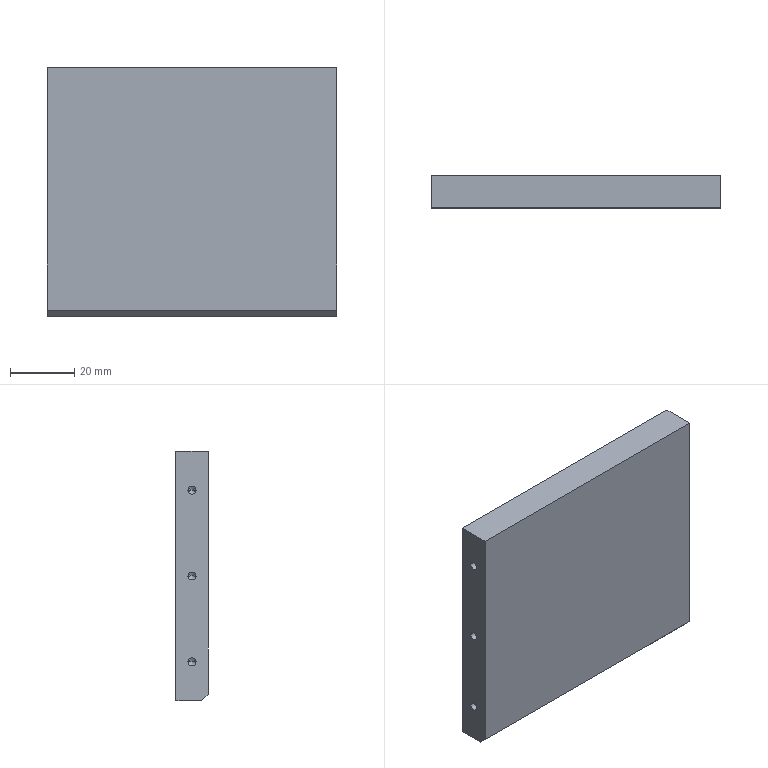Component | SolidWorks | 170423A4-SafetyPowerProbeFixingPlate4-1 | 1 solid | 31 faces | box 90 x 10 x 77.5 mm | volume 69312 mm3 | cylinder 12 | cone 12 | plane 7 | commonest cylinder face diameters 2.5 x12
build123d program:
from build123d import *

# Parameters (mm, degrees)
SKETCH1_W             = 90
SKETCH1_H             = 77.5
BOSS_EXTRUDE1_DEPTH   = 10
M3_TAPPED_HOLE1_D     = 2.5
M3_TAPPED_HOLE1_DEPTH = 8.5
M3_TAPPED_HOLE1_TIP   = 0.7511
M3_TAPPED_HOLE2_D     = 2.5
M3_TAPPED_HOLE2_DEPTH = 8.5
M3_TAPPED_HOLE2_TIP   = 0.7511
CHAMFER1_SIZE         = 2


with BuildPart() as part:
    # Sketch1 → Boss-Extrude1 (new body)
    with BuildSketch(Plane.XY):
        Rectangle(SKETCH1_W, SKETCH1_H)
    extrude(amount=BOSS_EXTRUDE1_DEPTH)

    # M3 Tapped Hole1
    with Locations(Plane(origin=(45, 0, 0), x_dir=(0, 0, -1), z_dir=(1, 0, 0))):
        with Locations((-5, 26.75), (-5, -26.75), (-5, 0)):
            Hole(M3_TAPPED_HOLE1_D / 2, depth=M3_TAPPED_HOLE1_DEPTH)
            with Locations((0, 0, -(M3_TAPPED_HOLE1_DEPTH + M3_TAPPED_HOLE1_TIP / 2))):  # 118° drill point
                Cone(0, M3_TAPPED_HOLE1_D / 2, M3_TAPPED_HOLE1_TIP, mode=Mode.SUBTRACT)

    # M3 Tapped Hole2
    with Locations(Plane.ZY.offset(45)):
        with Locations((5, 26.75), (5, 0), (5, -26.75)):
            Hole(M3_TAPPED_HOLE2_D / 2, depth=M3_TAPPED_HOLE2_DEPTH)
            with Locations((0, 0, -(M3_TAPPED_HOLE2_DEPTH + M3_TAPPED_HOLE2_TIP / 2))):  # 118° drill point
                Cone(0, M3_TAPPED_HOLE2_D / 2, M3_TAPPED_HOLE2_TIP, mode=Mode.SUBTRACT)

    # Chamfer1
    chamfer1_edges = [part.edges().sort_by_distance(p)[0] for p in [
        (0, 38.75, 10),
    ]]
    chamfer(chamfer1_edges, length=CHAMFER1_SIZE)


solid = part.part

# Placed as in the assembly
solid = solid.moved(Location((28.687, -15.611, -40.824), (90, 0, -180)))
STEP:
#1=CARTESIAN_POINT('',(2.566,-0.7622,-2.66));
#2=VERTEX_POINT('',#1);
#3=CARTESIAN_POINT('',(2.566,-0.8607,-2.66));
#4=VERTEX_POINT('',#3);
#5=CARTESIAN_POINT('',(2.566,-0.8115,-2.66));
#6=DIRECTION('',(1.,0.,0.));
#7=DIRECTION('',(0.,-1.,0.));
#8=AXIS2_PLACEMENT_3D('',#5,#6,#7);
#9=CIRCLE('',#8,0.04921);
#10=EDGE_CURVE('',#2,#4,#9,.T.);
#11=ORIENTED_EDGE('',*,*,#10,.F.);
#12=CARTESIAN_POINT('',(2.901,-0.7622,-2.66));
#13=VERTEX_POINT('',#12);
#14=CARTESIAN_POINT('',(2.901,-0.7622,-2.66));
#15=DIRECTION('',(1.,0.,0.));
#16=VECTOR('',#15,39.37);
#17=LINE('',#14,#16);
#18=EDGE_CURVE('',#2,#13,#17,.T.);
#19=ORIENTED_EDGE('',*,*,#18,.T.);
#20=CARTESIAN_POINT('',(2.901,-0.8607,-2.66));
#21=VERTEX_POINT('',#20);
#22=CARTESIAN_POINT('',(2.901,-0.8115,-2.66));
#23=DIRECTION('',(1.,0.,0.));
#24=DIRECTION('',(0.,-1.,0.));
#25=AXIS2_PLACEMENT_3D('',#22,#23,#24);
#26=CIRCLE('',#25,0.04921);
#27=EDGE_CURVE('',#13,#21,#26,.T.);
#28=ORIENTED_EDGE('',*,*,#27,.T.);
#29=CARTESIAN_POINT('',(2.901,-0.8607,-2.66));
#30=DIRECTION('',(1.,0.,0.));
#31=VECTOR('',#30,39.37);
#32=LINE('',#29,#31);
#33=EDGE_CURVE('',#4,#21,#32,.T.);
#34=ORIENTED_EDGE('',*,*,#33,.F.);
#35=EDGE_LOOP('',(#11,#19,#28,#34));
#36=FACE_OUTER_BOUND('',#35,.T.);
#37=CARTESIAN_POINT('',(2.901,-0.8115,-2.66));
#38=DIRECTION('',(1.,0.,0.));
#39=DIRECTION('',(0.,-1.,0.));
#40=AXIS2_PLACEMENT_3D('',#37,#38,#39);
#41=CYLINDRICAL_SURFACE('',#40,0.04921);
#42=ADVANCED_FACE('',(#36),#41,.F.);
#43=CARTESIAN_POINT('',(2.537,-0.8115,-2.66));
#44=VERTEX_POINT('',#43);
#45=CARTESIAN_POINT('',(2.566,-0.8607,-2.66));
#46=DIRECTION('',(0.515,-0.8572,0.));
#47=VECTOR('',#46,39.37);
#48=LINE('',#45,#47);
#49=EDGE_CURVE('',#44,#4,#48,.T.);
#50=ORIENTED_EDGE('',*,*,#49,.F.);
#51=CARTESIAN_POINT('',(2.566,-0.7622,-2.66));
#52=DIRECTION('',(0.515,0.8572,-0.));
#53=VECTOR('',#52,39.37);
#54=LINE('',#51,#53);
#55=EDGE_CURVE('',#44,#2,#54,.T.);
#56=ORIENTED_EDGE('',*,*,#55,.T.);
#57=ORIENTED_EDGE('',*,*,#10,.T.);
#58=EDGE_LOOP('',(#50,#56,#57));
#59=FACE_OUTER_BOUND('',#58,.T.);
#60=CARTESIAN_POINT('',(2.566,-0.8115,-2.66));
#61=DIRECTION('',(1.,0.,0.));
#62=DIRECTION('',(0.,-1.,0.));
#63=AXIS2_PLACEMENT_3D('',#60,#61,#62);
#64=CONICAL_SURFACE('',#63,0.04921,1.03);
#65=ADVANCED_FACE('',(#59),#64,.F.);
#66=CARTESIAN_POINT('',(2.566,-0.7622,-1.607));
#67=VERTEX_POINT('',#66);
#68=CARTESIAN_POINT('',(2.566,-0.8607,-1.607));
#69=VERTEX_POINT('',#68);
#70=CARTESIAN_POINT('',(2.566,-0.8115,-1.607));
#71=DIRECTION('',(1.,0.,0.));
#72=DIRECTION('',(0.,-1.,0.));
#73=AXIS2_PLACEMENT_3D('',#70,#71,#72);
#74=CIRCLE('',#73,0.04921);
#75=EDGE_CURVE('',#67,#69,#74,.T.);
#76=ORIENTED_EDGE('',*,*,#75,.F.);
#77=CARTESIAN_POINT('',(2.901,-0.7622,-1.607));
#78=VERTEX_POINT('',#77);
#79=CARTESIAN_POINT('',(2.901,-0.7622,-1.607));
#80=DIRECTION('',(1.,0.,0.));
#81=VECTOR('',#80,39.37);
#82=LINE('',#79,#81);
#83=EDGE_CURVE('',#67,#78,#82,.T.);
#84=ORIENTED_EDGE('',*,*,#83,.T.);
#85=CARTESIAN_POINT('',(2.901,-0.8607,-1.607));
#86=VERTEX_POINT('',#85);
#87=CARTESIAN_POINT('',(2.901,-0.8115,-1.607));
#88=DIRECTION('',(1.,0.,0.));
#89=DIRECTION('',(0.,-1.,0.));
#90=AXIS2_PLACEMENT_3D('',#87,#88,#89);
#91=CIRCLE('',#90,0.04921);
#92=EDGE_CURVE('',#78,#86,#91,.T.);
#93=ORIENTED_EDGE('',*,*,#92,.T.);
#94=CARTESIAN_POINT('',(2.901,-0.8607,-1.607));
#95=DIRECTION('',(1.,0.,0.));
#96=VECTOR('',#95,39.37);
#97=LINE('',#94,#96);
#98=EDGE_CURVE('',#69,#86,#97,.T.);
#99=ORIENTED_EDGE('',*,*,#98,.F.);
#100=EDGE_LOOP('',(#76,#84,#93,#99));
#101=FACE_OUTER_BOUND('',#100,.T.);
#102=CARTESIAN_POINT('',(2.901,-0.8115,-1.607));
#103=DIRECTION('',(1.,0.,0.));
#104=DIRECTION('',(0.,-1.,0.));
#105=AXIS2_PLACEMENT_3D('',#102,#103,#104);
#106=CYLINDRICAL_SURFACE('',#105,0.04921);
#107=ADVANCED_FACE('',(#101),#106,.F.);
#108=CARTESIAN_POINT('',(2.537,-0.8115,-1.607));
#109=VERTEX_POINT('',#108);
#110=CARTESIAN_POINT('',(2.566,-0.8607,-1.607));
#111=DIRECTION('',(0.515,-0.8572,0.));
#112=VECTOR('',#111,39.37);
#113=LINE('',#110,#112);
#114=EDGE_CURVE('',#109,#69,#113,.T.);
#115=ORIENTED_EDGE('',*,*,#114,.F.);
#116=CARTESIAN_POINT('',(2.566,-0.7622,-1.607));
#117=DIRECTION('',(0.515,0.8572,-0.));
#118=VECTOR('',#117,39.37);
#119=LINE('',#116,#118);
#120=EDGE_CURVE('',#109,#67,#119,.T.);
#121=ORIENTED_EDGE('',*,*,#120,.T.);
#122=ORIENTED_EDGE('',*,*,#75,.T.);
#123=EDGE_LOOP('',(#115,#121,#122));
#124=FACE_OUTER_BOUND('',#123,.T.);
#125=CARTESIAN_POINT('',(2.566,-0.8115,-1.607));
#126=DIRECTION('',(1.,0.,0.));
#127=DIRECTION('',(0.,-1.,0.));
#128=AXIS2_PLACEMENT_3D('',#125,#126,#127);
#129=CONICAL_SURFACE('',#128,0.04921,1.03);
#130=ADVANCED_FACE('',(#124),#129,.F.);
#131=CARTESIAN_POINT('',(2.566,-0.7622,-0.5541));
#132=VERTEX_POINT('',#131);
#133=CARTESIAN_POINT('',(2.566,-0.8607,-0.5541));
#134=VERTEX_POINT('',#133);
#135=CARTESIAN_POINT('',(2.566,-0.8115,-0.5541));
#136=DIRECTION('',(1.,0.,0.));
#137=DIRECTION('',(0.,-1.,0.));
#138=AXIS2_PLACEMENT_3D('',#135,#136,#137);
#139=CIRCLE('',#138,0.04921);
#140=EDGE_CURVE('',#132,#134,#139,.T.);
#141=ORIENTED_EDGE('',*,*,#140,.F.);
#142=CARTESIAN_POINT('',(2.901,-0.7622,-0.5541));
#143=VERTEX_POINT('',#142);
#144=CARTESIAN_POINT('',(2.901,-0.7622,-0.5541));
#145=DIRECTION('',(1.,0.,0.));
#146=VECTOR('',#145,39.37);
#147=LINE('',#144,#146);
#148=EDGE_CURVE('',#132,#143,#147,.T.);
#149=ORIENTED_EDGE('',*,*,#148,.T.);
#150=CARTESIAN_POINT('',(2.901,-0.8607,-0.5541));
#151=VERTEX_POINT('',#150);
#152=CARTESIAN_POINT('',(2.901,-0.8115,-0.5541));
#153=DIRECTION('',(1.,0.,0.));
#154=DIRECTION('',(0.,-1.,0.));
#155=AXIS2_PLACEMENT_3D('',#152,#153,#154);
#156=CIRCLE('',#155,0.04921);
#157=EDGE_CURVE('',#143,#151,#156,.T.);
#158=ORIENTED_EDGE('',*,*,#157,.T.);
#159=CARTESIAN_POINT('',(2.901,-0.8607,-0.5541));
#160=DIRECTION('',(1.,0.,0.));
#161=VECTOR('',#160,39.37);
#162=LINE('',#159,#161);
#163=EDGE_CURVE('',#134,#151,#162,.T.);
#164=ORIENTED_EDGE('',*,*,#163,.F.);
#165=EDGE_LOOP('',(#141,#149,#158,#164));
#166=FACE_OUTER_BOUND('',#165,.T.);
#167=CARTESIAN_POINT('',(2.901,-0.8115,-0.5541));
#168=DIRECTION('',(1.,0.,0.));
#169=DIRECTION('',(0.,-1.,0.));
#170=AXIS2_PLACEMENT_3D('',#167,#168,#169);
#171=CYLINDRICAL_SURFACE('',#170,0.04921);
#172=ADVANCED_FACE('',(#166),#171,.F.);
#173=CARTESIAN_POINT('',(2.537,-0.8115,-0.5541));
#174=VERTEX_POINT('',#173);
#175=CARTESIAN_POINT('',(2.566,-0.8607,-0.5541));
#176=DIRECTION('',(0.515,-0.8572,0.));
#177=VECTOR('',#176,39.37);
#178=LINE('',#175,#177);
#179=EDGE_CURVE('',#174,#134,#178,.T.);
#180=ORIENTED_EDGE('',*,*,#179,.F.);
#181=CARTESIAN_POINT('',(2.566,-0.7622,-0.5541));
#182=DIRECTION('',(0.515,0.8572,-0.));
#183=VECTOR('',#182,39.37);
#184=LINE('',#181,#183);
#185=EDGE_CURVE('',#174,#132,#184,.T.);
#186=ORIENTED_EDGE('',*,*,#185,.T.);
#187=ORIENTED_EDGE('',*,*,#140,.T.);
#188=EDGE_LOOP('',(#180,#186,#187));
#189=FACE_OUTER_BOUND('',#188,.T.);
#190=CARTESIAN_POINT('',(2.566,-0.8115,-0.5541));
#191=DIRECTION('',(1.,0.,0.));
#192=DIRECTION('',(0.,-1.,0.));
#193=AXIS2_PLACEMENT_3D('',#190,#191,#192);
#194=CONICAL_SURFACE('',#193,0.04921,1.03);
#195=ADVANCED_FACE('',(#189),#194,.F.);
#196=CARTESIAN_POINT('',(-0.3076,-0.8607,-0.5541));
#197=VERTEX_POINT('',#196);
#198=CARTESIAN_POINT('',(-0.3076,-0.7622,-0.5541));
#199=VERTEX_POINT('',#198);
#200=CARTESIAN_POINT('',(-0.3076,-0.8115,-0.5541));
#201=DIRECTION('',(-1.,-0.,-0.));
#202=DIRECTION('',(0.,1.,0.));
#203=AXIS2_PLACEMENT_3D('',#200,#201,#202);
#204=CIRCLE('',#203,0.04921);
#205=EDGE_CURVE('',#197,#199,#204,.T.);
#206=ORIENTED_EDGE('',*,*,#205,.F.);
#207=CARTESIAN_POINT('',(-0.6423,-0.8607,-0.5541));
#208=VERTEX_POINT('',#207);
#209=CARTESIAN_POINT('',(-0.6423,-0.8607,-0.5541));
#210=DIRECTION('',(-1.,-0.,-0.));
#211=VECTOR('',#210,39.37);
#212=LINE('',#209,#211);
#213=EDGE_CURVE('',#197,#208,#212,.T.);
#214=ORIENTED_EDGE('',*,*,#213,.T.);
#215=CARTESIAN_POINT('',(-0.6423,-0.7622,-0.5541));
#216=VERTEX_POINT('',#215);
#217=CARTESIAN_POINT('',(-0.6423,-0.8115,-0.5541));
#218=DIRECTION('',(-1.,-0.,-0.));
#219=DIRECTION('',(0.,1.,0.));
#220=AXIS2_PLACEMENT_3D('',#217,#218,#219);
#221=CIRCLE('',#220,0.04921);
#222=EDGE_CURVE('',#208,#216,#221,.T.);
#223=ORIENTED_EDGE('',*,*,#222,.T.);
#224=CARTESIAN_POINT('',(-0.6423,-0.7622,-0.5541));
#225=DIRECTION('',(-1.,-0.,-0.));
#226=VECTOR('',#225,39.37);
#227=LINE('',#224,#226);
#228=EDGE_CURVE('',#199,#216,#227,.T.);
#229=ORIENTED_EDGE('',*,*,#228,.F.);
#230=EDGE_LOOP('',(#206,#214,#223,#229));
#231=FACE_OUTER_BOUND('',#230,.T.);
#232=CARTESIAN_POINT('',(-0.6423,-0.8115,-0.5541));
#233=DIRECTION('',(-1.,-0.,-0.));
#234=DIRECTION('',(0.,1.,0.));
#235=AXIS2_PLACEMENT_3D('',#232,#233,#234);
#236=CYLINDRICAL_SURFACE('',#235,0.04921);
#237=ADVANCED_FACE('',(#231),#236,.F.);
#238=CARTESIAN_POINT('',(-0.278,-0.8115,-0.5541));
#239=VERTEX_POINT('',#238);
#240=CARTESIAN_POINT('',(-0.3076,-0.7622,-0.5541));
#241=DIRECTION('',(-0.515,0.8572,-0.));
#242=VECTOR('',#241,39.37);
#243=LINE('',#240,#242);
#244=EDGE_CURVE('',#239,#199,#243,.T.);
#245=ORIENTED_EDGE('',*,*,#244,.F.);
#246=CARTESIAN_POINT('',(-0.3076,-0.8607,-0.5541));
#247=DIRECTION('',(-0.515,-0.8572,-0.));
#248=VECTOR('',#247,39.37);
#249=LINE('',#246,#248);
#250=EDGE_CURVE('',#239,#197,#249,.T.);
#251=ORIENTED_EDGE('',*,*,#250,.T.);
#252=ORIENTED_EDGE('',*,*,#205,.T.);
#253=EDGE_LOOP('',(#245,#251,#252));
#254=FACE_OUTER_BOUND('',#253,.T.);
#255=CARTESIAN_POINT('',(-0.3076,-0.8115,-0.5541));
#256=DIRECTION('',(-1.,-0.,-0.));
#257=DIRECTION('',(0.,1.,0.));
#258=AXIS2_PLACEMENT_3D('',#255,#256,#257);
#259=CONICAL_SURFACE('',#258,0.04921,1.03);
#260=ADVANCED_FACE('',(#254),#259,.F.);
#261=CARTESIAN_POINT('',(-0.3076,-0.8607,-1.607));
#262=VERTEX_POINT('',#261);
#263=CARTESIAN_POINT('',(-0.3076,-0.7622,-1.607));
#264=VERTEX_POINT('',#263);
#265=CARTESIAN_POINT('',(-0.3076,-0.8115,-1.607));
#266=DIRECTION('',(-1.,-0.,-0.));
#267=DIRECTION('',(0.,1.,0.));
#268=AXIS2_PLACEMENT_3D('',#265,#266,#267);
#269=CIRCLE('',#268,0.04921);
#270=EDGE_CURVE('',#262,#264,#269,.T.);
#271=ORIENTED_EDGE('',*,*,#270,.F.);
#272=CARTESIAN_POINT('',(-0.6423,-0.8607,-1.607));
#273=VERTEX_POINT('',#272);
#274=CARTESIAN_POINT('',(-0.6423,-0.8607,-1.607));
#275=DIRECTION('',(-1.,-0.,-0.));
#276=VECTOR('',#275,39.37);
#277=LINE('',#274,#276);
#278=EDGE_CURVE('',#262,#273,#277,.T.);
#279=ORIENTED_EDGE('',*,*,#278,.T.);
#280=CARTESIAN_POINT('',(-0.6423,-0.7622,-1.607));
#281=VERTEX_POINT('',#280);
#282=CARTESIAN_POINT('',(-0.6423,-0.8115,-1.607));
#283=DIRECTION('',(-1.,-0.,-0.));
#284=DIRECTION('',(0.,1.,0.));
#285=AXIS2_PLACEMENT_3D('',#282,#283,#284);
#286=CIRCLE('',#285,0.04921);
#287=EDGE_CURVE('',#273,#281,#286,.T.);
#288=ORIENTED_EDGE('',*,*,#287,.T.);
#289=CARTESIAN_POINT('',(-0.6423,-0.7622,-1.607));
#290=DIRECTION('',(-1.,-0.,-0.));
#291=VECTOR('',#290,39.37);
#292=LINE('',#289,#291);
#293=EDGE_CURVE('',#264,#281,#292,.T.);
#294=ORIENTED_EDGE('',*,*,#293,.F.);
#295=EDGE_LOOP('',(#271,#279,#288,#294));
#296=FACE_OUTER_BOUND('',#295,.T.);
#297=CARTESIAN_POINT('',(-0.6423,-0.8115,-1.607));
#298=DIRECTION('',(-1.,-0.,-0.));
#299=DIRECTION('',(0.,1.,0.));
#300=AXIS2_PLACEMENT_3D('',#297,#298,#299);
#301=CYLINDRICAL_SURFACE('',#300,0.04921);
#302=ADVANCED_FACE('',(#296),#301,.F.);
#303=CARTESIAN_POINT('',(-0.278,-0.8115,-1.607));
#304=VERTEX_POINT('',#303);
#305=CARTESIAN_POINT('',(-0.3076,-0.7622,-1.607));
#306=DIRECTION('',(-0.515,0.8572,-0.));
#307=VECTOR('',#306,39.37);
#308=LINE('',#305,#307);
#309=EDGE_CURVE('',#304,#264,#308,.T.);
#310=ORIENTED_EDGE('',*,*,#309,.F.);
#311=CARTESIAN_POINT('',(-0.3076,-0.8607,-1.607));
#312=DIRECTION('',(-0.515,-0.8572,-0.));
#313=VECTOR('',#312,39.37);
#314=LINE('',#311,#313);
#315=EDGE_CURVE('',#304,#262,#314,.T.);
#316=ORIENTED_EDGE('',*,*,#315,.T.);
#317=ORIENTED_EDGE('',*,*,#270,.T.);
#318=EDGE_LOOP('',(#310,#316,#317));
#319=FACE_OUTER_BOUND('',#318,.T.);
#320=CARTESIAN_POINT('',(-0.3076,-0.8115,-1.607));
#321=DIRECTION('',(-1.,-0.,-0.));
#322=DIRECTION('',(0.,1.,0.));
#323=AXIS2_PLACEMENT_3D('',#320,#321,#322);
#324=CONICAL_SURFACE('',#323,0.04921,1.03);
#325=ADVANCED_FACE('',(#319),#324,.F.);
#326=CARTESIAN_POINT('',(-0.3076,-0.8607,-2.66));
#327=VERTEX_POINT('',#326);
#328=CARTESIAN_POINT('',(-0.3076,-0.7622,-2.66));
#329=VERTEX_POINT('',#328);
#330=CARTESIAN_POINT('',(-0.3076,-0.8115,-2.66));
#331=DIRECTION('',(-1.,-0.,-0.));
#332=DIRECTION('',(0.,1.,0.));
#333=AXIS2_PLACEMENT_3D('',#330,#331,#332);
#334=CIRCLE('',#333,0.04921);
#335=EDGE_CURVE('',#327,#329,#334,.T.);
#336=ORIENTED_EDGE('',*,*,#335,.F.);
#337=CARTESIAN_POINT('',(-0.6423,-0.8607,-2.66));
#338=VERTEX_POINT('',#337);
#339=CARTESIAN_POINT('',(-0.6423,-0.8607,-2.66));
#340=DIRECTION('',(-1.,-0.,-0.));
#341=VECTOR('',#340,39.37);
#342=LINE('',#339,#341);
#343=EDGE_CURVE('',#327,#338,#342,.T.);
#344=ORIENTED_EDGE('',*,*,#343,.T.);
#345=CARTESIAN_POINT('',(-0.6423,-0.7622,-2.66));
#346=VERTEX_POINT('',#345);
#347=CARTESIAN_POINT('',(-0.6423,-0.8115,-2.66));
#348=DIRECTION('',(-1.,-0.,-0.));
#349=DIRECTION('',(0.,1.,0.));
#350=AXIS2_PLACEMENT_3D('',#347,#348,#349);
#351=CIRCLE('',#350,0.04921);
#352=EDGE_CURVE('',#338,#346,#351,.T.);
#353=ORIENTED_EDGE('',*,*,#352,.T.);
#354=CARTESIAN_POINT('',(-0.6423,-0.7622,-2.66));
#355=DIRECTION('',(-1.,-0.,-0.));
#356=VECTOR('',#355,39.37);
#357=LINE('',#354,#356);
#358=EDGE_CURVE('',#329,#346,#357,.T.);
#359=ORIENTED_EDGE('',*,*,#358,.F.);
#360=EDGE_LOOP('',(#336,#344,#353,#359));
#361=FACE_OUTER_BOUND('',#360,.T.);
#362=CARTESIAN_POINT('',(-0.6423,-0.8115,-2.66));
#363=DIRECTION('',(-1.,-0.,-0.));
#364=DIRECTION('',(0.,1.,0.));
#365=AXIS2_PLACEMENT_3D('',#362,#363,#364);
#366=CYLINDRICAL_SURFACE('',#365,0.04921);
#367=ADVANCED_FACE('',(#361),#366,.F.);
#368=CARTESIAN_POINT('',(-0.278,-0.8115,-2.66));
#369=VERTEX_POINT('',#368);
#370=CARTESIAN_POINT('',(-0.3076,-0.7622,-2.66));
#371=DIRECTION('',(-0.515,0.8572,-0.));
#372=VECTOR('',#371,39.37);
#373=LINE('',#370,#372);
#374=EDGE_CURVE('',#369,#329,#373,.T.);
#375=ORIENTED_EDGE('',*,*,#374,.F.);
#376=CARTESIAN_POINT('',(-0.3076,-0.8607,-2.66));
#377=DIRECTION('',(-0.515,-0.8572,-0.));
#378=VECTOR('',#377,39.37);
#379=LINE('',#376,#378);
#380=EDGE_CURVE('',#369,#327,#379,.T.);
#381=ORIENTED_EDGE('',*,*,#380,.T.);
#382=ORIENTED_EDGE('',*,*,#335,.T.);
#383=EDGE_LOOP('',(#375,#381,#382));
#384=FACE_OUTER_BOUND('',#383,.T.);
#385=CARTESIAN_POINT('',(-0.3076,-0.8115,-2.66));
#386=DIRECTION('',(-1.,-0.,-0.));
#387=DIRECTION('',(0.,1.,0.));
#388=AXIS2_PLACEMENT_3D('',#385,#386,#387);
#389=CONICAL_SURFACE('',#388,0.04921,1.03);
#390=ADVANCED_FACE('',(#384),#389,.F.);
#391=CARTESIAN_POINT('',(-0.6423,-0.8115,-0.5541));
#392=DIRECTION('',(-1.,-0.,-0.));
#393=DIRECTION('',(0.,1.,0.));
#394=AXIS2_PLACEMENT_3D('',#391,#392,#393);
#395=CIRCLE('',#394,0.04921);
#396=EDGE_CURVE('',#216,#208,#395,.T.);
#397=ORIENTED_EDGE('',*,*,#396,.F.);
#398=ORIENTED_EDGE('',*,*,#222,.F.);
#399=EDGE_LOOP('',(#397,#398));
#400=FACE_BOUND('',#399,.T.);
#401=CARTESIAN_POINT('',(-0.6423,-0.8115,-1.607));
#402=DIRECTION('',(-1.,-0.,-0.));
#403=DIRECTION('',(0.,1.,0.));
#404=AXIS2_PLACEMENT_3D('',#401,#402,#403);
#405=CIRCLE('',#404,0.04921);
#406=EDGE_CURVE('',#281,#273,#405,.T.);
#407=ORIENTED_EDGE('',*,*,#406,.F.);
#408=ORIENTED_EDGE('',*,*,#287,.F.);
#409=EDGE_LOOP('',(#407,#408));
#410=FACE_BOUND('',#409,.T.);
#411=CARTESIAN_POINT('',(-0.6423,-0.8115,-2.66));
#412=DIRECTION('',(-1.,-0.,-0.));
#413=DIRECTION('',(0.,1.,0.));
#414=AXIS2_PLACEMENT_3D('',#411,#412,#413);
#415=CIRCLE('',#414,0.04921);
#416=EDGE_CURVE('',#346,#338,#415,.T.);
#417=ORIENTED_EDGE('',*,*,#416,.F.);
#418=ORIENTED_EDGE('',*,*,#352,.F.);
#419=EDGE_LOOP('',(#417,#418));
#420=FACE_BOUND('',#419,.T.);
#421=CARTESIAN_POINT('',(-0.6423,-0.9296,-3.133));
#422=VERTEX_POINT('',#421);
#423=CARTESIAN_POINT('',(-0.6423,-0.6146,-3.133));
#424=VERTEX_POINT('',#423);
#425=CARTESIAN_POINT('',(-0.6423,-1.008,-3.133));
#426=DIRECTION('',(-0.,1.,0.));
#427=VECTOR('',#426,39.37);
#428=LINE('',#425,#427);
#429=EDGE_CURVE('',#422,#424,#428,.T.);
#430=ORIENTED_EDGE('',*,*,#429,.F.);
#431=CARTESIAN_POINT('',(-0.6423,-1.008,-3.054));
#432=VERTEX_POINT('',#431);
#433=CARTESIAN_POINT('',(-0.6423,-1.008,-3.054));
#434=DIRECTION('',(-0.,-0.7071,0.7071));
#435=VECTOR('',#434,39.37);
#436=LINE('',#433,#435);
#437=EDGE_CURVE('',#422,#432,#436,.T.);
#438=ORIENTED_EDGE('',*,*,#437,.T.);
#439=CARTESIAN_POINT('',(-0.6423,-1.008,-0.08165));
#440=VERTEX_POINT('',#439);
#441=CARTESIAN_POINT('',(-0.6423,-1.008,-3.133));
#442=DIRECTION('',(0.,-0.,-1.));
#443=VECTOR('',#442,39.37);
#444=LINE('',#441,#443);
#445=EDGE_CURVE('',#440,#432,#444,.T.);
#446=ORIENTED_EDGE('',*,*,#445,.F.);
#447=CARTESIAN_POINT('',(-0.6423,-0.6146,-0.08165));
#448=VERTEX_POINT('',#447);
#449=CARTESIAN_POINT('',(-0.6423,-1.008,-0.08165));
#450=DIRECTION('',(-0.,1.,0.));
#451=VECTOR('',#450,39.37);
#452=LINE('',#449,#451);
#453=EDGE_CURVE('',#440,#448,#452,.T.);
#454=ORIENTED_EDGE('',*,*,#453,.T.);
#455=CARTESIAN_POINT('',(-0.6423,-0.6146,-3.133));
#456=DIRECTION('',(0.,-0.,-1.));
#457=VECTOR('',#456,39.37);
#458=LINE('',#455,#457);
#459=EDGE_CURVE('',#448,#424,#458,.T.);
#460=ORIENTED_EDGE('',*,*,#459,.T.);
#461=EDGE_LOOP('',(#430,#438,#446,#454,#460));
#462=FACE_OUTER_BOUND('',#461,.T.);
#463=CARTESIAN_POINT('',(-0.6423,-1.008,-3.133));
#464=DIRECTION('',(1.,0.,0.));
#465=DIRECTION('',(-0.,0.,1.));
#466=AXIS2_PLACEMENT_3D('',#463,#464,#465);
#467=PLANE('',#466);
#468=ADVANCED_FACE('',(#400,#410,#420,#462),#467,.F.);
#469=CARTESIAN_POINT('',(2.901,-0.9296,-3.133));
#470=VERTEX_POINT('',#469);
#471=CARTESIAN_POINT('',(2.901,-0.6146,-3.133));
#472=VERTEX_POINT('',#471);
#473=CARTESIAN_POINT('',(2.901,-1.008,-3.133));
#474=DIRECTION('',(-0.,1.,0.));
#475=VECTOR('',#474,39.37);
#476=LINE('',#473,#475);
#477=EDGE_CURVE('',#470,#472,#476,.T.);
#478=ORIENTED_EDGE('',*,*,#477,.F.);
#479=CARTESIAN_POINT('',(-0.6423,-0.9296,-3.133));
#480=DIRECTION('',(-1.,-0.,-0.));
#481=VECTOR('',#480,39.37);
#482=LINE('',#479,#481);
#483=EDGE_CURVE('',#470,#422,#482,.T.);
#484=ORIENTED_EDGE('',*,*,#483,.T.);
#485=ORIENTED_EDGE('',*,*,#429,.T.);
#486=CARTESIAN_POINT('',(2.901,-0.6146,-3.133));
#487=DIRECTION('',(1.,0.,0.));
#488=VECTOR('',#487,39.37);
#489=LINE('',#486,#488);
#490=EDGE_CURVE('',#424,#472,#489,.T.);
#491=ORIENTED_EDGE('',*,*,#490,.T.);
#492=EDGE_LOOP('',(#478,#484,#485,#491));
#493=FACE_OUTER_BOUND('',#492,.T.);
#494=CARTESIAN_POINT('',(2.901,-1.008,-3.133));
#495=DIRECTION('',(0.,-0.,1.));
#496=DIRECTION('',(-0.,1.,0.));
#497=AXIS2_PLACEMENT_3D('',#494,#495,#496);
#498=PLANE('',#497);
#499=ADVANCED_FACE('',(#493),#498,.F.);
#500=CARTESIAN_POINT('',(2.901,-0.8115,-2.66));
#501=DIRECTION('',(1.,0.,0.));
#502=DIRECTION('',(0.,-1.,0.));
#503=AXIS2_PLACEMENT_3D('',#500,#501,#502);
#504=CIRCLE('',#503,0.04921);
#505=EDGE_CURVE('',#21,#13,#504,.T.);
#506=ORIENTED_EDGE('',*,*,#505,.F.);
#507=ORIENTED_EDGE('',*,*,#27,.F.);
#508=EDGE_LOOP('',(#506,#507));
#509=FACE_BOUND('',#508,.T.);
#510=CARTESIAN_POINT('',(2.901,-0.8115,-1.607));
#511=DIRECTION('',(1.,0.,0.));
#512=DIRECTION('',(0.,-1.,0.));
#513=AXIS2_PLACEMENT_3D('',#510,#511,#512);
#514=CIRCLE('',#513,0.04921);
#515=EDGE_CURVE('',#86,#78,#514,.T.);
#516=ORIENTED_EDGE('',*,*,#515,.F.);
#517=ORIENTED_EDGE('',*,*,#92,.F.);
#518=EDGE_LOOP('',(#516,#517));
#519=FACE_BOUND('',#518,.T.);
#520=CARTESIAN_POINT('',(2.901,-0.8115,-0.5541));
#521=DIRECTION('',(1.,0.,0.));
#522=DIRECTION('',(0.,-1.,0.));
#523=AXIS2_PLACEMENT_3D('',#520,#521,#522);
#524=CIRCLE('',#523,0.04921);
#525=EDGE_CURVE('',#151,#143,#524,.T.);
#526=ORIENTED_EDGE('',*,*,#525,.F.);
#527=ORIENTED_EDGE('',*,*,#157,.F.);
#528=EDGE_LOOP('',(#526,#527));
#529=FACE_BOUND('',#528,.T.);
#530=CARTESIAN_POINT('',(2.901,-1.008,-3.054));
#531=VERTEX_POINT('',#530);
#532=CARTESIAN_POINT('',(2.901,-1.008,-0.08165));
#533=VERTEX_POINT('',#532);
#534=CARTESIAN_POINT('',(2.901,-1.008,-3.133));
#535=DIRECTION('',(-0.,0.,1.));
#536=VECTOR('',#535,39.37);
#537=LINE('',#534,#536);
#538=EDGE_CURVE('',#531,#533,#537,.T.);
#539=ORIENTED_EDGE('',*,*,#538,.F.);
#540=CARTESIAN_POINT('',(2.901,-1.008,-3.054));
#541=DIRECTION('',(-0.,0.7071,-0.7071));
#542=VECTOR('',#541,39.37);
#543=LINE('',#540,#542);
#544=EDGE_CURVE('',#531,#470,#543,.T.);
#545=ORIENTED_EDGE('',*,*,#544,.T.);
#546=ORIENTED_EDGE('',*,*,#477,.T.);
#547=CARTESIAN_POINT('',(2.901,-0.6146,-0.08165));
#548=VERTEX_POINT('',#547);
#549=CARTESIAN_POINT('',(2.901,-0.6146,-3.133));
#550=DIRECTION('',(-0.,0.,1.));
#551=VECTOR('',#550,39.37);
#552=LINE('',#549,#551);
#553=EDGE_CURVE('',#472,#548,#552,.T.);
#554=ORIENTED_EDGE('',*,*,#553,.T.);
#555=CARTESIAN_POINT('',(2.901,-1.008,-0.08165));
#556=DIRECTION('',(-0.,1.,0.));
#557=VECTOR('',#556,39.37);
#558=LINE('',#555,#557);
#559=EDGE_CURVE('',#533,#548,#558,.T.);
#560=ORIENTED_EDGE('',*,*,#559,.F.);
#561=EDGE_LOOP('',(#539,#545,#546,#554,#560));
#562=FACE_OUTER_BOUND('',#561,.T.);
#563=CARTESIAN_POINT('',(2.901,-1.008,-3.133));
#564=DIRECTION('',(-1.,-0.,-0.));
#565=DIRECTION('',(0.,-0.,-1.));
#566=AXIS2_PLACEMENT_3D('',#563,#564,#565);
#567=PLANE('',#566);
#568=ADVANCED_FACE('',(#509,#519,#529,#562),#567,.F.);
#569=CARTESIAN_POINT('',(2.901,-0.6146,-0.08165));
#570=DIRECTION('',(-1.,-0.,-0.));
#571=VECTOR('',#570,39.37);
#572=LINE('',#569,#571);
#573=EDGE_CURVE('',#548,#448,#572,.T.);
#574=ORIENTED_EDGE('',*,*,#573,.T.);
#575=ORIENTED_EDGE('',*,*,#453,.F.);
#576=CARTESIAN_POINT('',(2.901,-1.008,-0.08165));
#577=DIRECTION('',(-1.,-0.,-0.));
#578=VECTOR('',#577,39.37);
#579=LINE('',#576,#578);
#580=EDGE_CURVE('',#533,#440,#579,.T.);
#581=ORIENTED_EDGE('',*,*,#580,.F.);
#582=ORIENTED_EDGE('',*,*,#559,.T.);
#583=EDGE_LOOP('',(#574,#575,#581,#582));
#584=FACE_OUTER_BOUND('',#583,.T.);
#585=CARTESIAN_POINT('',(2.901,-1.008,-0.08165));
#586=DIRECTION('',(-0.,0.,-1.));
#587=DIRECTION('',(0.,-1.,-0.));
#588=AXIS2_PLACEMENT_3D('',#585,#586,#587);
#589=PLANE('',#588);
#590=ADVANCED_FACE('',(#584),#589,.F.);
#591=ORIENTED_EDGE('',*,*,#445,.T.);
#592=CARTESIAN_POINT('',(2.901,-1.008,-3.054));
#593=DIRECTION('',(1.,0.,0.));
#594=VECTOR('',#593,39.37);
#595=LINE('',#592,#594);
#596=EDGE_CURVE('',#432,#531,#595,.T.);
#597=ORIENTED_EDGE('',*,*,#596,.T.);
#598=ORIENTED_EDGE('',*,*,#538,.T.);
#599=ORIENTED_EDGE('',*,*,#580,.T.);
#600=EDGE_LOOP('',(#591,#597,#598,#599));
#601=FACE_OUTER_BOUND('',#600,.T.);
#602=CARTESIAN_POINT('',(1.129,-1.008,-1.607));
#603=DIRECTION('',(0.,-1.,-0.));
#604=DIRECTION('',(-1.,-0.,-0.));
#605=AXIS2_PLACEMENT_3D('',#602,#603,#604);
#606=PLANE('',#605);
#607=ADVANCED_FACE('',(#601),#606,.T.);
#608=ORIENTED_EDGE('',*,*,#459,.F.);
#609=ORIENTED_EDGE('',*,*,#573,.F.);
#610=ORIENTED_EDGE('',*,*,#553,.F.);
#611=ORIENTED_EDGE('',*,*,#490,.F.);
#612=EDGE_LOOP('',(#608,#609,#610,#611));
#613=FACE_OUTER_BOUND('',#612,.T.);
#614=CARTESIAN_POINT('',(1.129,-0.6146,-1.607));
#615=DIRECTION('',(0.,-1.,-0.));
#616=DIRECTION('',(-1.,-0.,-0.));
#617=AXIS2_PLACEMENT_3D('',#614,#615,#616);
#618=PLANE('',#617);
#619=ADVANCED_FACE('',(#613),#618,.F.);
#620=ORIENTED_EDGE('',*,*,#380,.F.);
#621=ORIENTED_EDGE('',*,*,#374,.T.);
#622=CARTESIAN_POINT('',(-0.3076,-0.8115,-2.66));
#623=DIRECTION('',(-1.,-0.,-0.));
#624=DIRECTION('',(0.,1.,0.));
#625=AXIS2_PLACEMENT_3D('',#622,#623,#624);
#626=CIRCLE('',#625,0.04921);
#627=EDGE_CURVE('',#329,#327,#626,.T.);
#628=ORIENTED_EDGE('',*,*,#627,.T.);
#629=EDGE_LOOP('',(#620,#621,#628));
#630=FACE_OUTER_BOUND('',#629,.T.);
#631=CARTESIAN_POINT('',(-0.3076,-0.8115,-2.66));
#632=DIRECTION('',(-1.,-0.,-0.));
#633=DIRECTION('',(0.,1.,0.));
#634=AXIS2_PLACEMENT_3D('',#631,#632,#633);
#635=CONICAL_SURFACE('',#634,0.04921,1.03);
#636=ADVANCED_FACE('',(#630),#635,.F.);
#637=ORIENTED_EDGE('',*,*,#343,.F.);
#638=ORIENTED_EDGE('',*,*,#627,.F.);
#639=ORIENTED_EDGE('',*,*,#358,.T.);
#640=ORIENTED_EDGE('',*,*,#416,.T.);
#641=EDGE_LOOP('',(#637,#638,#639,#640));
#642=FACE_OUTER_BOUND('',#641,.T.);
#643=CARTESIAN_POINT('',(-0.6423,-0.8115,-2.66));
#644=DIRECTION('',(-1.,-0.,-0.));
#645=DIRECTION('',(0.,1.,0.));
#646=AXIS2_PLACEMENT_3D('',#643,#644,#645);
#647=CYLINDRICAL_SURFACE('',#646,0.04921);
#648=ADVANCED_FACE('',(#642),#647,.F.);
#649=ORIENTED_EDGE('',*,*,#315,.F.);
#650=ORIENTED_EDGE('',*,*,#309,.T.);
#651=CARTESIAN_POINT('',(-0.3076,-0.8115,-1.607));
#652=DIRECTION('',(-1.,-0.,-0.));
#653=DIRECTION('',(0.,1.,0.));
#654=AXIS2_PLACEMENT_3D('',#651,#652,#653);
#655=CIRCLE('',#654,0.04921);
#656=EDGE_CURVE('',#264,#262,#655,.T.);
#657=ORIENTED_EDGE('',*,*,#656,.T.);
#658=EDGE_LOOP('',(#649,#650,#657));
#659=FACE_OUTER_BOUND('',#658,.T.);
#660=CARTESIAN_POINT('',(-0.3076,-0.8115,-1.607));
#661=DIRECTION('',(-1.,-0.,-0.));
#662=DIRECTION('',(0.,1.,0.));
#663=AXIS2_PLACEMENT_3D('',#660,#661,#662);
#664=CONICAL_SURFACE('',#663,0.04921,1.03);
#665=ADVANCED_FACE('',(#659),#664,.F.);
#666=ORIENTED_EDGE('',*,*,#278,.F.);
#667=ORIENTED_EDGE('',*,*,#656,.F.);
#668=ORIENTED_EDGE('',*,*,#293,.T.);
#669=ORIENTED_EDGE('',*,*,#406,.T.);
#670=EDGE_LOOP('',(#666,#667,#668,#669));
#671=FACE_OUTER_BOUND('',#670,.T.);
#672=CARTESIAN_POINT('',(-0.6423,-0.8115,-1.607));
#673=DIRECTION('',(-1.,-0.,-0.));
#674=DIRECTION('',(0.,1.,0.));
#675=AXIS2_PLACEMENT_3D('',#672,#673,#674);
#676=CYLINDRICAL_SURFACE('',#675,0.04921);
#677=ADVANCED_FACE('',(#671),#676,.F.);
#678=ORIENTED_EDGE('',*,*,#250,.F.);
#679=ORIENTED_EDGE('',*,*,#244,.T.);
#680=CARTESIAN_POINT('',(-0.3076,-0.8115,-0.5541));
#681=DIRECTION('',(-1.,-0.,-0.));
#682=DIRECTION('',(0.,1.,0.));
#683=AXIS2_PLACEMENT_3D('',#680,#681,#682);
#684=CIRCLE('',#683,0.04921);
#685=EDGE_CURVE('',#199,#197,#684,.T.);
#686=ORIENTED_EDGE('',*,*,#685,.T.);
#687=EDGE_LOOP('',(#678,#679,#686));
#688=FACE_OUTER_BOUND('',#687,.T.);
#689=CARTESIAN_POINT('',(-0.3076,-0.8115,-0.5541));
#690=DIRECTION('',(-1.,-0.,-0.));
#691=DIRECTION('',(0.,1.,0.));
#692=AXIS2_PLACEMENT_3D('',#689,#690,#691);
#693=CONICAL_SURFACE('',#692,0.04921,1.03);
#694=ADVANCED_FACE('',(#688),#693,.F.);
#695=ORIENTED_EDGE('',*,*,#213,.F.);
#696=ORIENTED_EDGE('',*,*,#685,.F.);
#697=ORIENTED_EDGE('',*,*,#228,.T.);
#698=ORIENTED_EDGE('',*,*,#396,.T.);
#699=EDGE_LOOP('',(#695,#696,#697,#698));
#700=FACE_OUTER_BOUND('',#699,.T.);
#701=CARTESIAN_POINT('',(-0.6423,-0.8115,-0.5541));
#702=DIRECTION('',(-1.,-0.,-0.));
#703=DIRECTION('',(0.,1.,0.));
#704=AXIS2_PLACEMENT_3D('',#701,#702,#703);
#705=CYLINDRICAL_SURFACE('',#704,0.04921);
#706=ADVANCED_FACE('',(#700),#705,.F.);
#707=ORIENTED_EDGE('',*,*,#185,.F.);
#708=ORIENTED_EDGE('',*,*,#179,.T.);
#709=CARTESIAN_POINT('',(2.566,-0.8115,-0.5541));
#710=DIRECTION('',(1.,0.,0.));
#711=DIRECTION('',(0.,-1.,0.));
#712=AXIS2_PLACEMENT_3D('',#709,#710,#711);
#713=CIRCLE('',#712,0.04921);
#714=EDGE_CURVE('',#134,#132,#713,.T.);
#715=ORIENTED_EDGE('',*,*,#714,.T.);
#716=EDGE_LOOP('',(#707,#708,#715));
#717=FACE_OUTER_BOUND('',#716,.T.);
#718=CARTESIAN_POINT('',(2.566,-0.8115,-0.5541));
#719=DIRECTION('',(1.,0.,0.));
#720=DIRECTION('',(0.,-1.,0.));
#721=AXIS2_PLACEMENT_3D('',#718,#719,#720);
#722=CONICAL_SURFACE('',#721,0.04921,1.03);
#723=ADVANCED_FACE('',(#717),#722,.F.);
#724=ORIENTED_EDGE('',*,*,#148,.F.);
#725=ORIENTED_EDGE('',*,*,#714,.F.);
#726=ORIENTED_EDGE('',*,*,#163,.T.);
#727=ORIENTED_EDGE('',*,*,#525,.T.);
#728=EDGE_LOOP('',(#724,#725,#726,#727));
#729=FACE_OUTER_BOUND('',#728,.T.);
#730=CARTESIAN_POINT('',(2.901,-0.8115,-0.5541));
#731=DIRECTION('',(1.,0.,0.));
#732=DIRECTION('',(0.,-1.,0.));
#733=AXIS2_PLACEMENT_3D('',#730,#731,#732);
#734=CYLINDRICAL_SURFACE('',#733,0.04921);
#735=ADVANCED_FACE('',(#729),#734,.F.);
#736=ORIENTED_EDGE('',*,*,#120,.F.);
#737=ORIENTED_EDGE('',*,*,#114,.T.);
#738=CARTESIAN_POINT('',(2.566,-0.8115,-1.607));
#739=DIRECTION('',(1.,0.,0.));
#740=DIRECTION('',(0.,-1.,0.));
#741=AXIS2_PLACEMENT_3D('',#738,#739,#740);
#742=CIRCLE('',#741,0.04921);
#743=EDGE_CURVE('',#69,#67,#742,.T.);
#744=ORIENTED_EDGE('',*,*,#743,.T.);
#745=EDGE_LOOP('',(#736,#737,#744));
#746=FACE_OUTER_BOUND('',#745,.T.);
#747=CARTESIAN_POINT('',(2.566,-0.8115,-1.607));
#748=DIRECTION('',(1.,0.,0.));
#749=DIRECTION('',(0.,-1.,0.));
#750=AXIS2_PLACEMENT_3D('',#747,#748,#749);
#751=CONICAL_SURFACE('',#750,0.04921,1.03);
#752=ADVANCED_FACE('',(#746),#751,.F.);
#753=ORIENTED_EDGE('',*,*,#83,.F.);
#754=ORIENTED_EDGE('',*,*,#743,.F.);
#755=ORIENTED_EDGE('',*,*,#98,.T.);
#756=ORIENTED_EDGE('',*,*,#515,.T.);
#757=EDGE_LOOP('',(#753,#754,#755,#756));
#758=FACE_OUTER_BOUND('',#757,.T.);
#759=CARTESIAN_POINT('',(2.901,-0.8115,-1.607));
#760=DIRECTION('',(1.,0.,0.));
#761=DIRECTION('',(0.,-1.,0.));
#762=AXIS2_PLACEMENT_3D('',#759,#760,#761);
#763=CYLINDRICAL_SURFACE('',#762,0.04921);
#764=ADVANCED_FACE('',(#758),#763,.F.);
#765=ORIENTED_EDGE('',*,*,#55,.F.);
#766=ORIENTED_EDGE('',*,*,#49,.T.);
#767=CARTESIAN_POINT('',(2.566,-0.8115,-2.66));
#768=DIRECTION('',(1.,0.,0.));
#769=DIRECTION('',(0.,-1.,0.));
#770=AXIS2_PLACEMENT_3D('',#767,#768,#769);
#771=CIRCLE('',#770,0.04921);
#772=EDGE_CURVE('',#4,#2,#771,.T.);
#773=ORIENTED_EDGE('',*,*,#772,.T.);
#774=EDGE_LOOP('',(#765,#766,#773));
#775=FACE_OUTER_BOUND('',#774,.T.);
#776=CARTESIAN_POINT('',(2.566,-0.8115,-2.66));
#777=DIRECTION('',(1.,0.,0.));
#778=DIRECTION('',(0.,-1.,0.));
#779=AXIS2_PLACEMENT_3D('',#776,#777,#778);
#780=CONICAL_SURFACE('',#779,0.04921,1.03);
#781=ADVANCED_FACE('',(#775),#780,.F.);
#782=ORIENTED_EDGE('',*,*,#18,.F.);
#783=ORIENTED_EDGE('',*,*,#772,.F.);
#784=ORIENTED_EDGE('',*,*,#33,.T.);
#785=ORIENTED_EDGE('',*,*,#505,.T.);
#786=EDGE_LOOP('',(#782,#783,#784,#785));
#787=FACE_OUTER_BOUND('',#786,.T.);
#788=CARTESIAN_POINT('',(2.901,-0.8115,-2.66));
#789=DIRECTION('',(1.,0.,0.));
#790=DIRECTION('',(0.,-1.,0.));
#791=AXIS2_PLACEMENT_3D('',#788,#789,#790);
#792=CYLINDRICAL_SURFACE('',#791,0.04921);
#793=ADVANCED_FACE('',(#787),#792,.F.);
#794=ORIENTED_EDGE('',*,*,#437,.F.);
#795=ORIENTED_EDGE('',*,*,#483,.F.);
#796=ORIENTED_EDGE('',*,*,#544,.F.);
#797=ORIENTED_EDGE('',*,*,#596,.F.);
#798=EDGE_LOOP('',(#794,#795,#796,#797));
#799=FACE_OUTER_BOUND('',#798,.T.);
#800=CARTESIAN_POINT('',(1.129,-1.008,-3.054));
#801=DIRECTION('',(0.,-0.7071,-0.7071));
#802=DIRECTION('',(-1.,-0.,-0.));
#803=AXIS2_PLACEMENT_3D('',#800,#801,#802);
#804=PLANE('',#803);
#805=ADVANCED_FACE('',(#799),#804,.T.);
#806=CLOSED_SHELL('',(#42,#65,#107,#130,#172,#195,#237,#260,#302,#325,#367,#390,#468,#499,#568,#590,#607,#619,#636,#648,#665,#677,#694,#706,#723,#735,#752,#764,#781,#793,#805));
#807=MANIFOLD_SOLID_BREP('',#806);
#808=CARTESIAN_POINT('',(0.,0.,0.));
#809=DIRECTION('',(0.,0.,1.));
#810=DIRECTION('',(1.,0.,0.));
#811=AXIS2_PLACEMENT_3D('',#808,#809,#810);
#812=(LENGTH_UNIT()NAMED_UNIT(*)SI_UNIT($,.METRE.));
#813=LENGTH_MEASURE_WITH_UNIT(LENGTH_MEASURE(0.0254),#812);
#814=DIMENSIONAL_EXPONENTS(1.,0.,0.,0.,0.,0.,0.);
#815=(CONVERSION_BASED_UNIT('',#813)LENGTH_UNIT()NAMED_UNIT(#814));
#816=UNCERTAINTY_MEASURE_WITH_UNIT(LENGTH_MEASURE(0.00001),#815,'','');
#817=(NAMED_UNIT(*)PLANE_ANGLE_UNIT()SI_UNIT($,.RADIAN.));
#818=(NAMED_UNIT(*)SI_UNIT($,.STERADIAN.)SOLID_ANGLE_UNIT());
#819=(GEOMETRIC_REPRESENTATION_CONTEXT(3)GLOBAL_UNCERTAINTY_ASSIGNED_CONTEXT((#816))GLOBAL_UNIT_ASSIGNED_CONTEXT((#815,#817,#818))REPRESENTATION_CONTEXT('',''));
#820=ADVANCED_BREP_SHAPE_REPRESENTATION('',(#807,#811),#819);
#821=COLOUR_RGB('',0.7922,0.8196,0.9333);
#822=FILL_AREA_STYLE_COLOUR('',#821);
#823=FILL_AREA_STYLE('',(#822));
#824=SURFACE_STYLE_FILL_AREA(#823);
#825=SURFACE_SIDE_STYLE('',(#824));
#826=SURFACE_STYLE_USAGE(.BOTH.,#825);
#827=PRESENTATION_STYLE_ASSIGNMENT((#826));
#828=STYLED_ITEM('',(#827),#807);
#829=PRESENTATION_LAYER_ASSIGNMENT('','',(#828));
#830=(LENGTH_UNIT()NAMED_UNIT(*)SI_UNIT($,.METRE.));
#831=LENGTH_MEASURE_WITH_UNIT(LENGTH_MEASURE(0.0254),#830);
#832=DIMENSIONAL_EXPONENTS(1.,0.,0.,0.,0.,0.,0.);
#833=(CONVERSION_BASED_UNIT('',#831)LENGTH_UNIT()NAMED_UNIT(#832));
#834=UNCERTAINTY_MEASURE_WITH_UNIT(LENGTH_MEASURE(0.00001),#833,'','');
#835=(NAMED_UNIT(*)PLANE_ANGLE_UNIT()SI_UNIT($,.RADIAN.));
#836=(NAMED_UNIT(*)SI_UNIT($,.STERADIAN.)SOLID_ANGLE_UNIT());
#837=(GEOMETRIC_REPRESENTATION_CONTEXT(3)GLOBAL_UNCERTAINTY_ASSIGNED_CONTEXT((#834))GLOBAL_UNIT_ASSIGNED_CONTEXT((#833,#835,#836))REPRESENTATION_CONTEXT('',''));
#838=MECHANICAL_DESIGN_GEOMETRIC_PRESENTATION_REPRESENTATION('',(#828),#837);